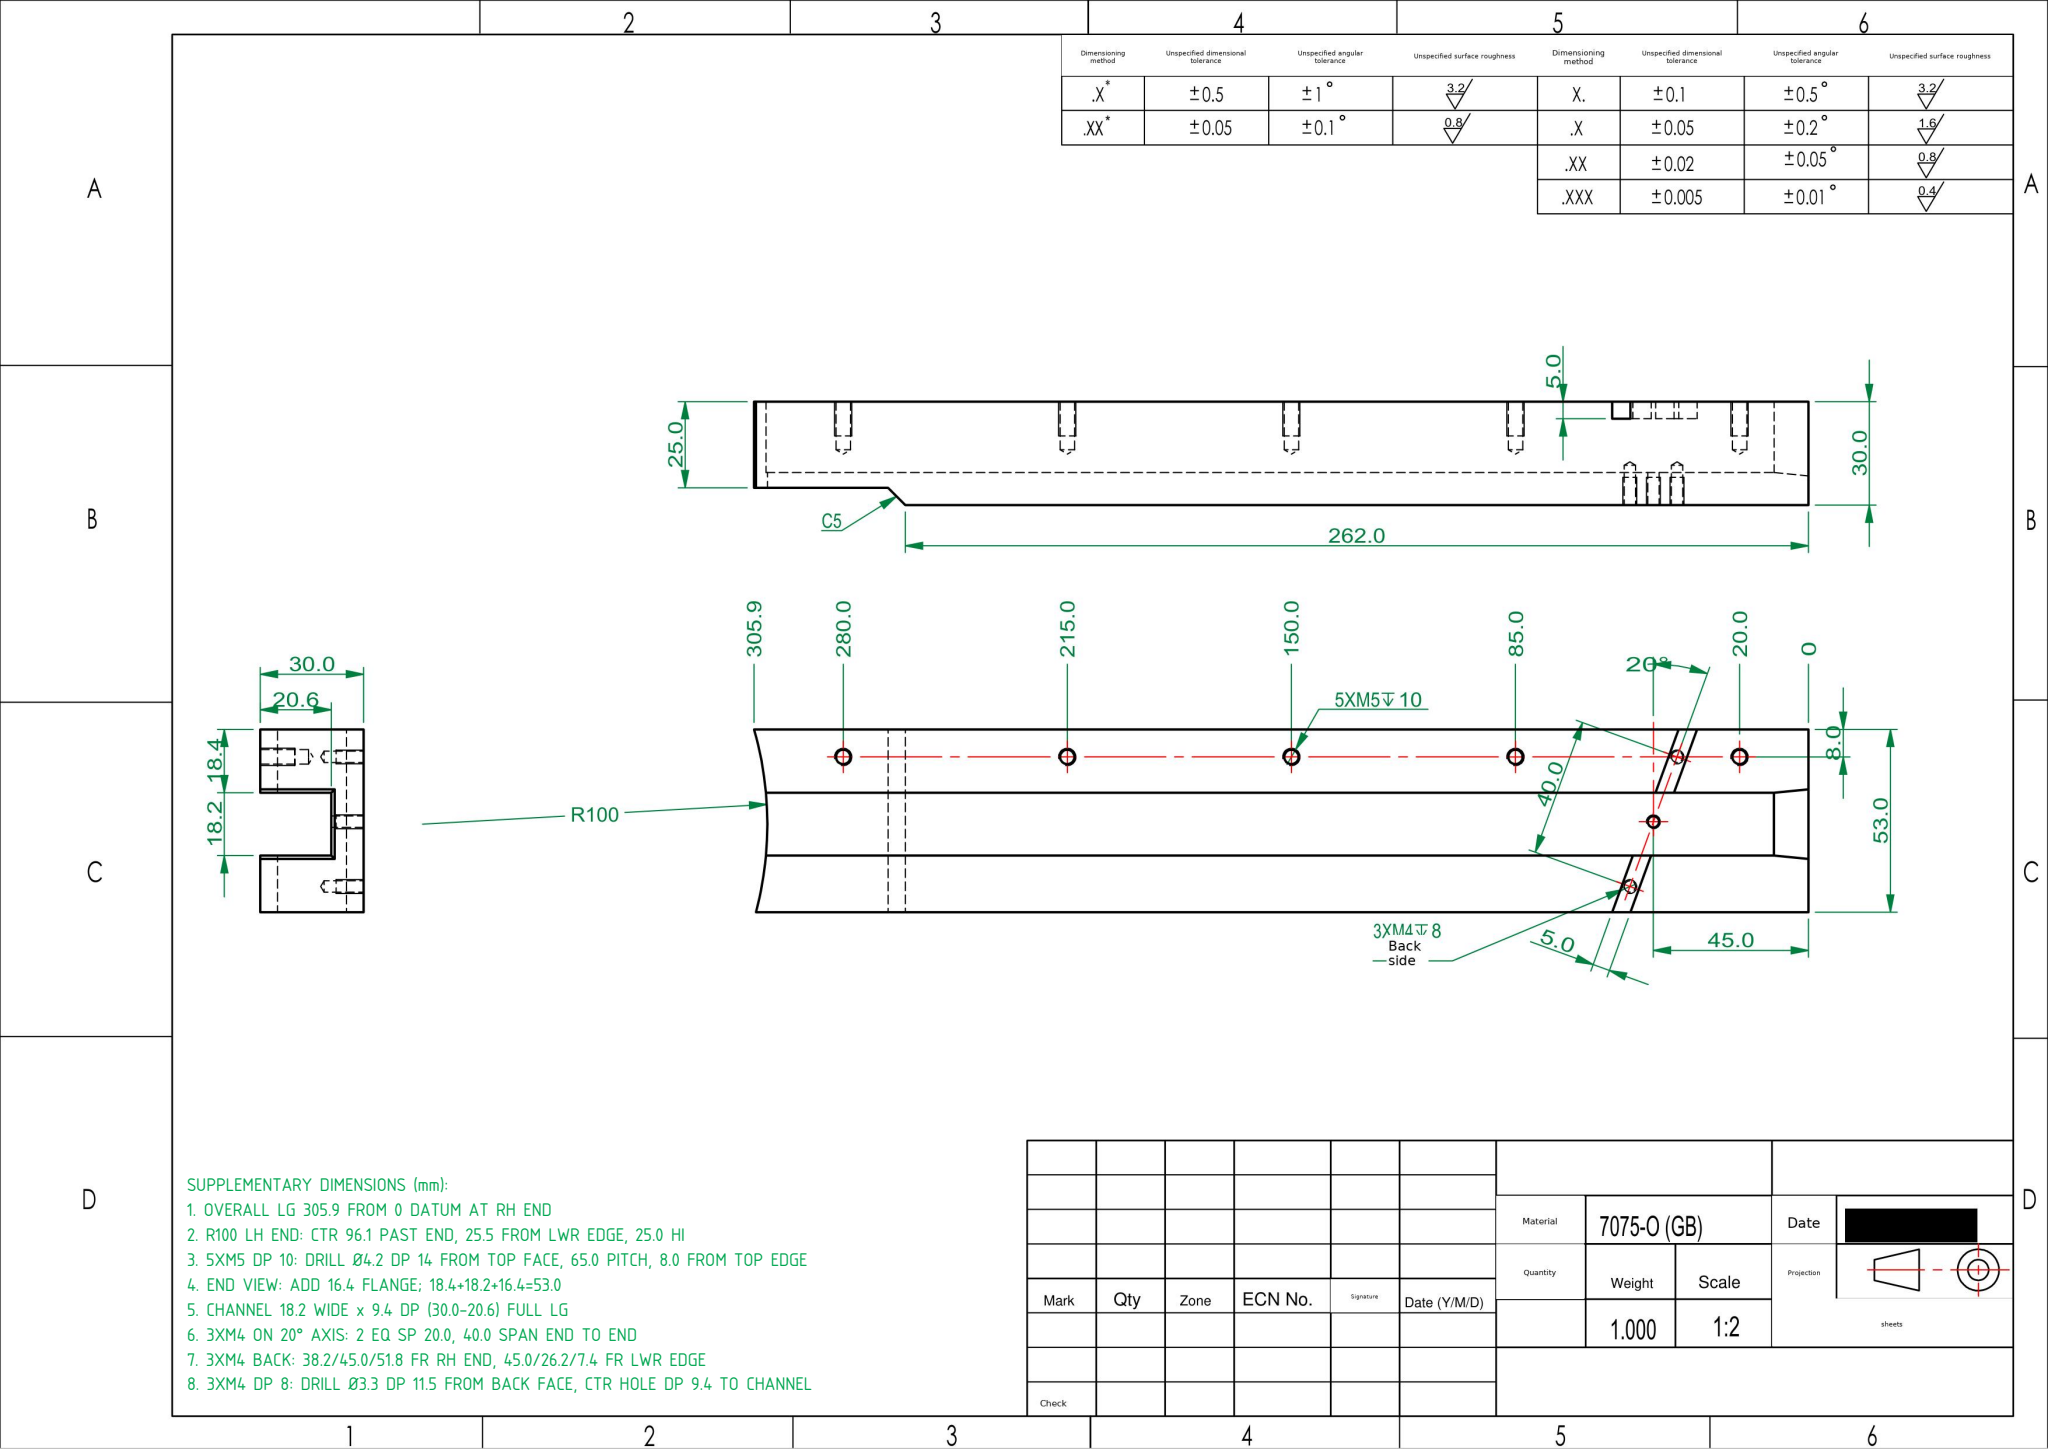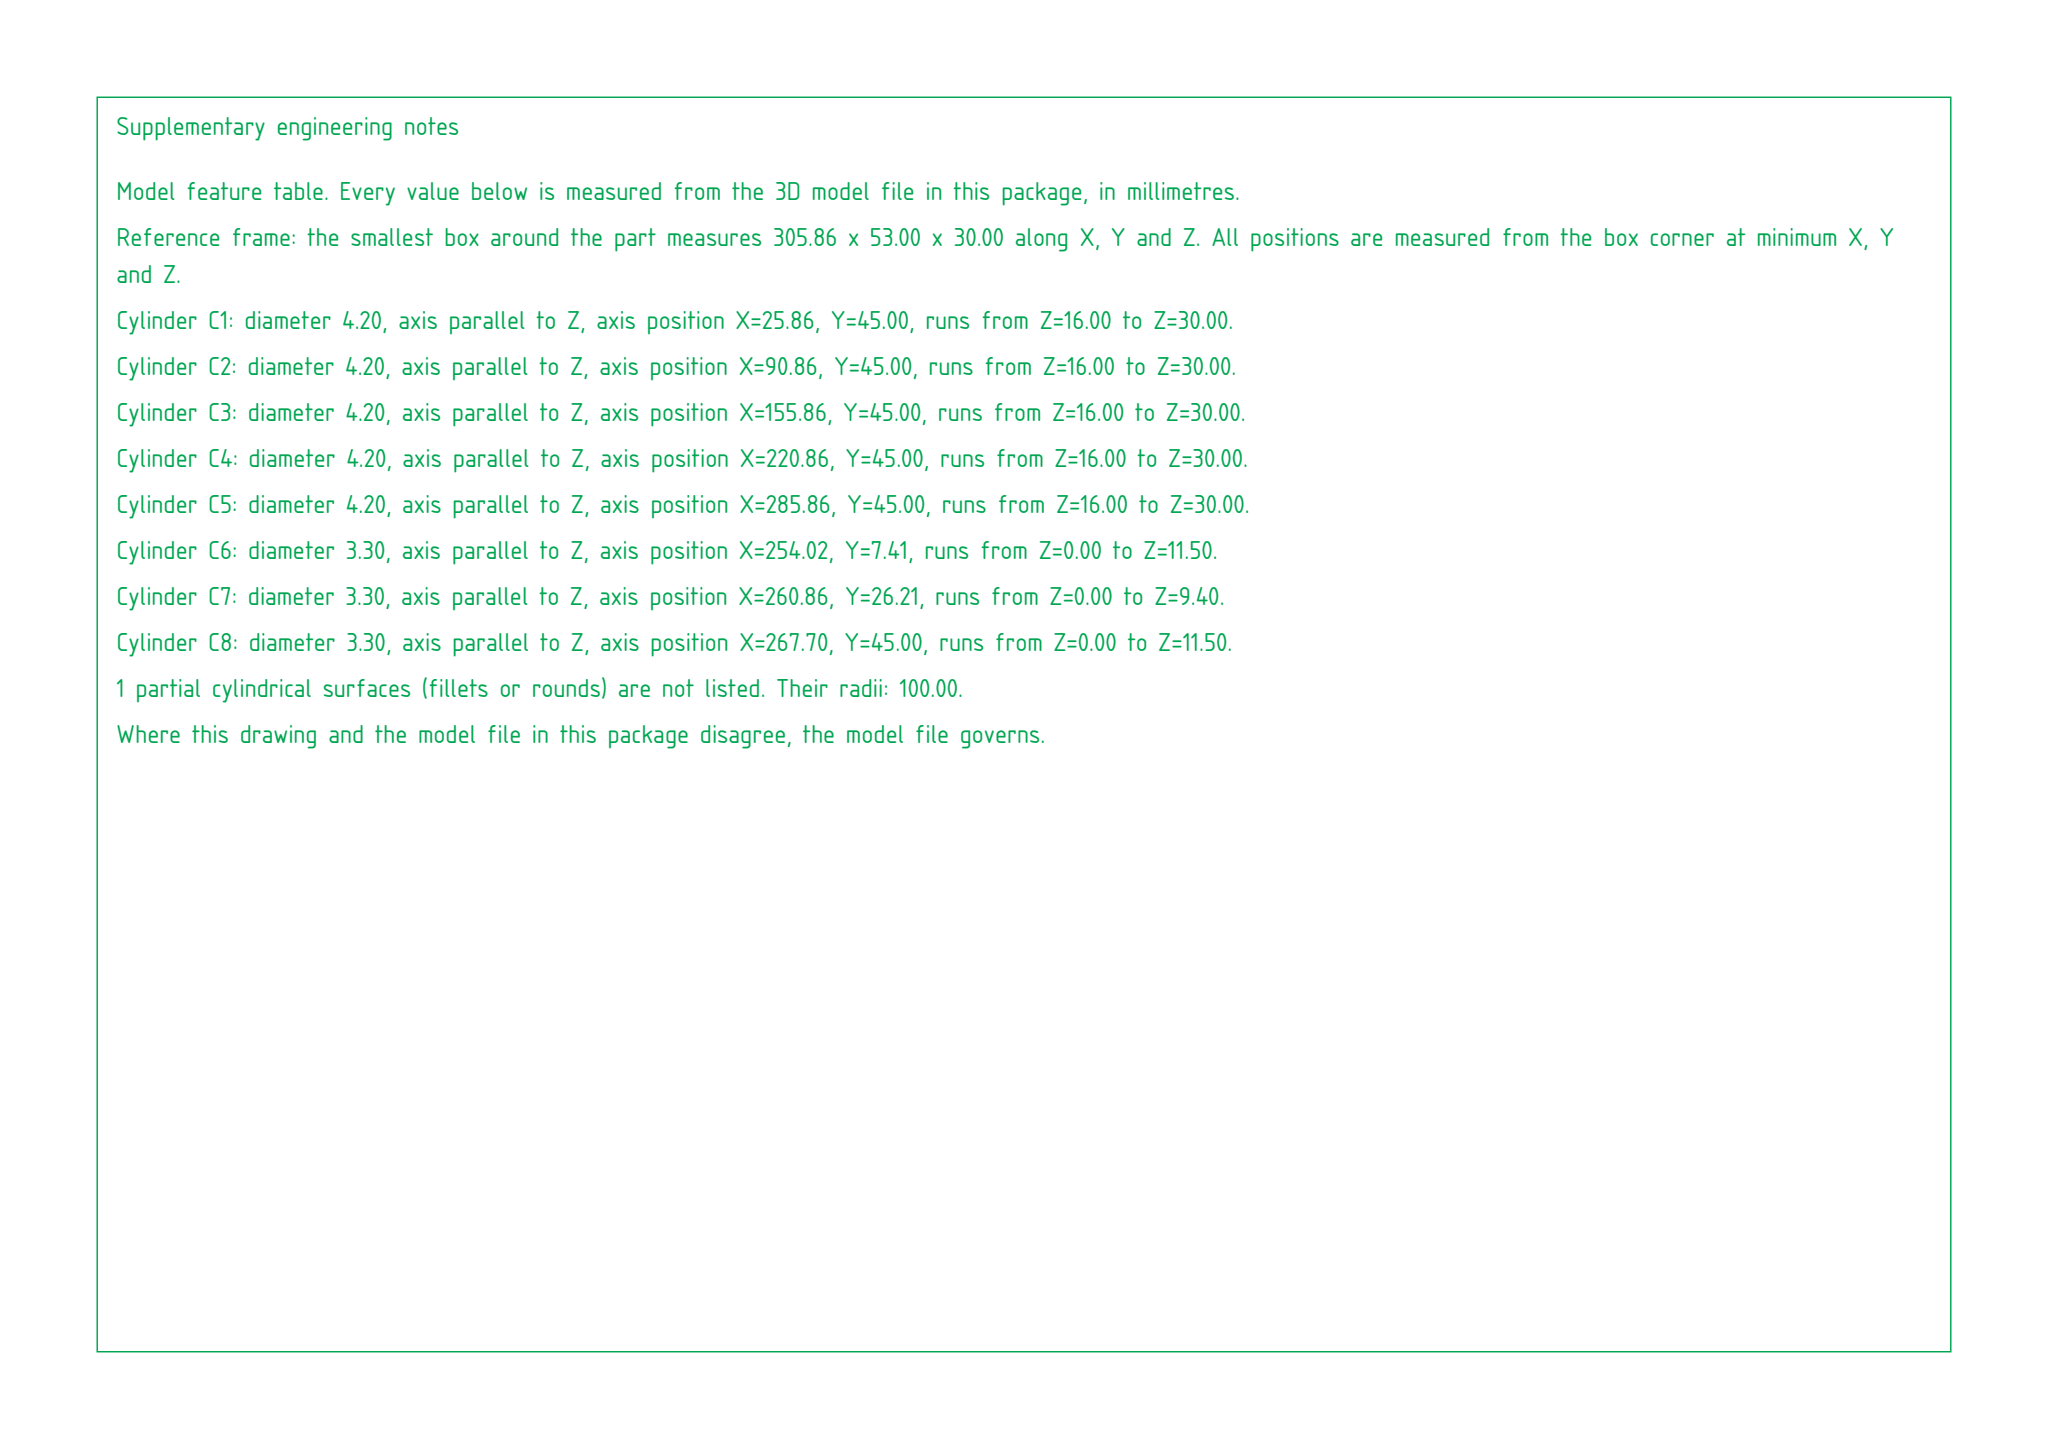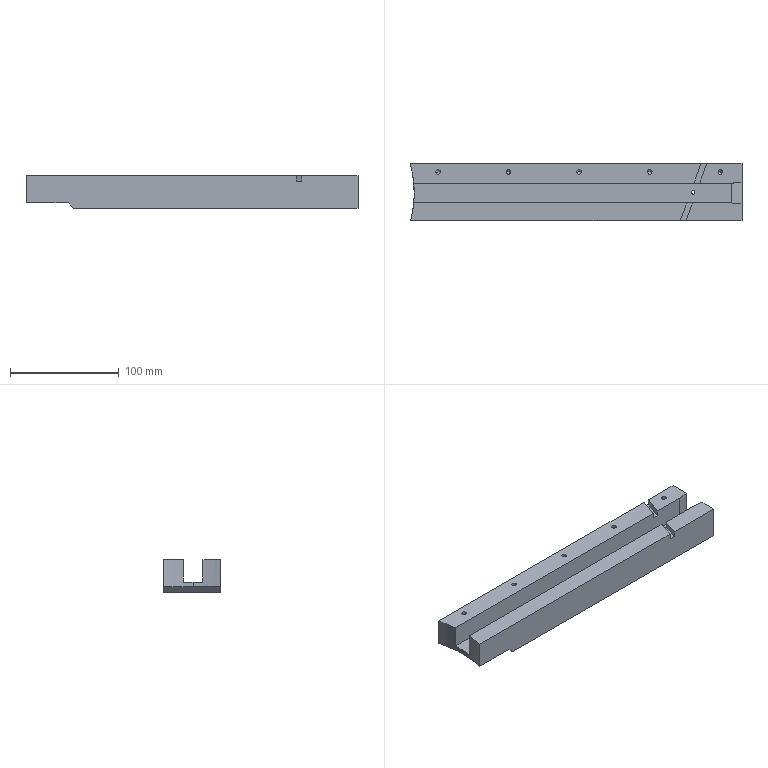Part | SolidWorks | mm | 1 solid | 54 faces | box 305.86 x 53 x 30 mm | volume 356028 mm3 | plane 22 | cylinder 18 | cone 14 | commonest cylinder face diameters 4.2 x10 3.3 x6 200 x2